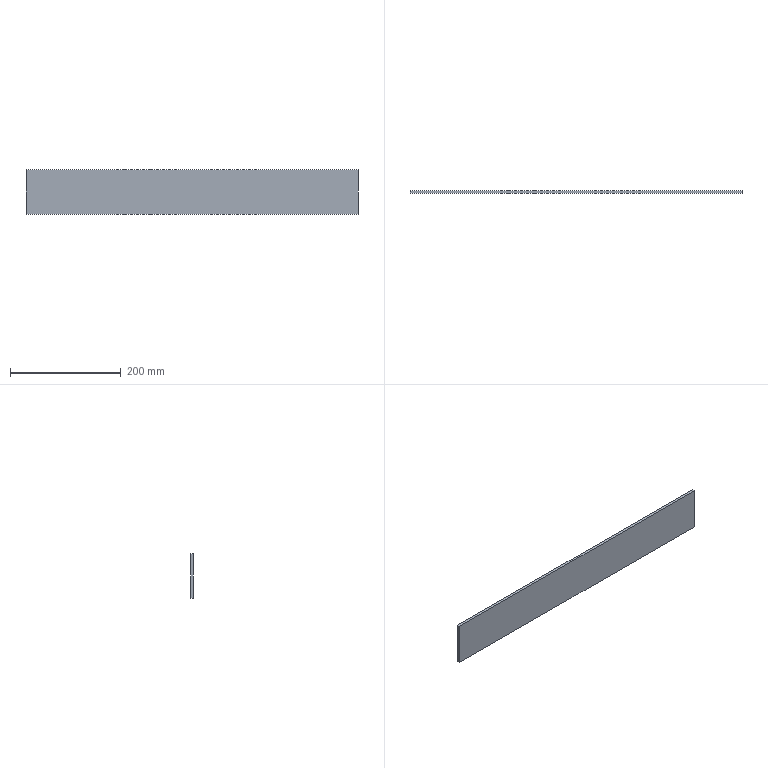Component | SolidWorks | CoverPlate6-1 | 1 solid | 6 faces | box 600 x 5 x 80 mm | volume 240000 mm3 | plane 6
build123d program:
from build123d import *

# Parameters (mm, degrees)
SKETCH1_W      = 600
SKETCH1_H      = 80
EXTRUDE1_DEPTH = 5


with BuildPart() as part:
    # Sketch1 → Extrude1 (new body)
    with BuildSketch(Plane.XY):
        Rectangle(SKETCH1_W, SKETCH1_H)
    extrude(amount=EXTRUDE1_DEPTH)


solid = part.part

# Placed as in the assembly
solid = solid.moved(Location((15, 95, -60), (90, 0, 0)))
STEP:
#1=COLOUR_RGB('',0.7922,0.8196,0.9333);
#2=FILL_AREA_STYLE_COLOUR('',#1);
#3=FILL_AREA_STYLE('',(#2));
#4=SURFACE_STYLE_FILL_AREA(#3);
#5=SURFACE_SIDE_STYLE('',(#4));
#6=SURFACE_STYLE_USAGE(.BOTH.,#5);
#7=PRESENTATION_STYLE_ASSIGNMENT((#6));
#8=CARTESIAN_POINT('',(12.402,3.543,-0.7874));
#9=VERTEX_POINT('',#8);
#10=CARTESIAN_POINT('',(12.402,3.543,-3.937));
#11=VERTEX_POINT('',#10);
#12=CARTESIAN_POINT('',(12.402,3.543,-3.937));
#13=DIRECTION('',(0.,0.,-1.));
#14=VECTOR('',#13,39.37);
#15=LINE('',#12,#14);
#16=EDGE_CURVE('',#9,#11,#15,.T.);
#17=ORIENTED_EDGE('',*,*,#16,.T.);
#18=CARTESIAN_POINT('',(12.402,3.74,-3.937));
#19=VERTEX_POINT('',#18);
#20=CARTESIAN_POINT('',(12.402,3.74,-3.937));
#21=DIRECTION('',(0.,-1.,0.));
#22=VECTOR('',#21,39.37);
#23=LINE('',#20,#22);
#24=EDGE_CURVE('',#19,#11,#23,.T.);
#25=ORIENTED_EDGE('',*,*,#24,.F.);
#26=CARTESIAN_POINT('',(12.402,3.74,-0.7874));
#27=VERTEX_POINT('',#26);
#28=CARTESIAN_POINT('',(12.402,3.74,-3.937));
#29=DIRECTION('',(0.,0.,-1.));
#30=VECTOR('',#29,39.37);
#31=LINE('',#28,#30);
#32=EDGE_CURVE('',#27,#19,#31,.T.);
#33=ORIENTED_EDGE('',*,*,#32,.F.);
#34=CARTESIAN_POINT('',(12.402,3.74,-0.7874));
#35=DIRECTION('',(0.,-1.,0.));
#36=VECTOR('',#35,39.37);
#37=LINE('',#34,#36);
#38=EDGE_CURVE('',#27,#9,#37,.T.);
#39=ORIENTED_EDGE('',*,*,#38,.T.);
#40=EDGE_LOOP('',(#17,#25,#33,#39));
#41=FACE_OUTER_BOUND('',#40,.T.);
#42=CARTESIAN_POINT('',(12.402,3.74,-3.937));
#43=DIRECTION('',(-1.,0.,0.));
#44=DIRECTION('',(0.,1.,0.));
#45=AXIS2_PLACEMENT_3D('',#42,#43,#44);
#46=PLANE('',#45);
#47=ADVANCED_FACE('',(#41),#46,.F.);
#48=CARTESIAN_POINT('',(-11.22,3.543,-3.937));
#49=VERTEX_POINT('',#48);
#50=CARTESIAN_POINT('',(-11.22,3.543,-3.937));
#51=DIRECTION('',(-1.,0.,0.));
#52=VECTOR('',#51,39.37);
#53=LINE('',#50,#52);
#54=EDGE_CURVE('',#11,#49,#53,.T.);
#55=ORIENTED_EDGE('',*,*,#54,.T.);
#56=CARTESIAN_POINT('',(-11.22,3.74,-3.937));
#57=VERTEX_POINT('',#56);
#58=CARTESIAN_POINT('',(-11.22,3.74,-3.937));
#59=DIRECTION('',(0.,-1.,0.));
#60=VECTOR('',#59,39.37);
#61=LINE('',#58,#60);
#62=EDGE_CURVE('',#57,#49,#61,.T.);
#63=ORIENTED_EDGE('',*,*,#62,.F.);
#64=CARTESIAN_POINT('',(-11.22,3.74,-3.937));
#65=DIRECTION('',(-1.,0.,0.));
#66=VECTOR('',#65,39.37);
#67=LINE('',#64,#66);
#68=EDGE_CURVE('',#19,#57,#67,.T.);
#69=ORIENTED_EDGE('',*,*,#68,.F.);
#70=ORIENTED_EDGE('',*,*,#24,.T.);
#71=EDGE_LOOP('',(#55,#63,#69,#70));
#72=FACE_OUTER_BOUND('',#71,.T.);
#73=CARTESIAN_POINT('',(-11.22,3.74,-3.937));
#74=DIRECTION('',(0.,0.,1.));
#75=DIRECTION('',(0.,-1.,0.));
#76=AXIS2_PLACEMENT_3D('',#73,#74,#75);
#77=PLANE('',#76);
#78=ADVANCED_FACE('',(#72),#77,.F.);
#79=CARTESIAN_POINT('',(-11.22,3.543,-0.7874));
#80=VERTEX_POINT('',#79);
#81=CARTESIAN_POINT('',(-11.22,3.543,-3.937));
#82=DIRECTION('',(0.,0.,1.));
#83=VECTOR('',#82,39.37);
#84=LINE('',#81,#83);
#85=EDGE_CURVE('',#49,#80,#84,.T.);
#86=ORIENTED_EDGE('',*,*,#85,.T.);
#87=CARTESIAN_POINT('',(-11.22,3.74,-0.7874));
#88=VERTEX_POINT('',#87);
#89=CARTESIAN_POINT('',(-11.22,3.74,-0.7874));
#90=DIRECTION('',(0.,-1.,0.));
#91=VECTOR('',#90,39.37);
#92=LINE('',#89,#91);
#93=EDGE_CURVE('',#88,#80,#92,.T.);
#94=ORIENTED_EDGE('',*,*,#93,.F.);
#95=CARTESIAN_POINT('',(-11.22,3.74,-3.937));
#96=DIRECTION('',(0.,0.,1.));
#97=VECTOR('',#96,39.37);
#98=LINE('',#95,#97);
#99=EDGE_CURVE('',#57,#88,#98,.T.);
#100=ORIENTED_EDGE('',*,*,#99,.F.);
#101=ORIENTED_EDGE('',*,*,#62,.T.);
#102=EDGE_LOOP('',(#86,#94,#100,#101));
#103=FACE_OUTER_BOUND('',#102,.T.);
#104=CARTESIAN_POINT('',(-11.22,3.74,-3.937));
#105=DIRECTION('',(1.,0.,0.));
#106=DIRECTION('',(0.,-1.,0.));
#107=AXIS2_PLACEMENT_3D('',#104,#105,#106);
#108=PLANE('',#107);
#109=ADVANCED_FACE('',(#103),#108,.F.);
#110=CARTESIAN_POINT('',(-11.22,3.543,-0.7874));
#111=DIRECTION('',(1.,0.,0.));
#112=VECTOR('',#111,39.37);
#113=LINE('',#110,#112);
#114=EDGE_CURVE('',#80,#9,#113,.T.);
#115=ORIENTED_EDGE('',*,*,#114,.T.);
#116=ORIENTED_EDGE('',*,*,#38,.F.);
#117=CARTESIAN_POINT('',(-11.22,3.74,-0.7874));
#118=DIRECTION('',(1.,0.,0.));
#119=VECTOR('',#118,39.37);
#120=LINE('',#117,#119);
#121=EDGE_CURVE('',#88,#27,#120,.T.);
#122=ORIENTED_EDGE('',*,*,#121,.F.);
#123=ORIENTED_EDGE('',*,*,#93,.T.);
#124=EDGE_LOOP('',(#115,#116,#122,#123));
#125=FACE_OUTER_BOUND('',#124,.T.);
#126=CARTESIAN_POINT('',(-11.22,3.74,-0.7874));
#127=DIRECTION('',(0.,0.,-1.));
#128=DIRECTION('',(0.,1.,0.));
#129=AXIS2_PLACEMENT_3D('',#126,#127,#128);
#130=PLANE('',#129);
#131=ADVANCED_FACE('',(#125),#130,.F.);
#132=ORIENTED_EDGE('',*,*,#32,.T.);
#133=ORIENTED_EDGE('',*,*,#68,.T.);
#134=ORIENTED_EDGE('',*,*,#99,.T.);
#135=ORIENTED_EDGE('',*,*,#121,.T.);
#136=EDGE_LOOP('',(#132,#133,#134,#135));
#137=FACE_OUTER_BOUND('',#136,.T.);
#138=CARTESIAN_POINT('',(0.5906,3.74,-2.362));
#139=DIRECTION('',(0.,1.,0.));
#140=DIRECTION('',(1.,0.,0.));
#141=AXIS2_PLACEMENT_3D('',#138,#139,#140);
#142=PLANE('',#141);
#143=ADVANCED_FACE('',(#137),#142,.T.);
#144=ORIENTED_EDGE('',*,*,#16,.F.);
#145=ORIENTED_EDGE('',*,*,#114,.F.);
#146=ORIENTED_EDGE('',*,*,#85,.F.);
#147=ORIENTED_EDGE('',*,*,#54,.F.);
#148=EDGE_LOOP('',(#144,#145,#146,#147));
#149=FACE_OUTER_BOUND('',#148,.T.);
#150=CARTESIAN_POINT('',(0.5906,3.543,-2.362));
#151=DIRECTION('',(0.,1.,0.));
#152=DIRECTION('',(1.,0.,0.));
#153=AXIS2_PLACEMENT_3D('',#150,#151,#152);
#154=PLANE('',#153);
#155=ADVANCED_FACE('',(#149),#154,.F.);
#156=CLOSED_SHELL('',(#47,#78,#109,#131,#143,#155));
#157=MANIFOLD_SOLID_BREP('',#156);
#158=STYLED_ITEM('',(#7),#157);
#159=(LENGTH_UNIT()NAMED_UNIT(*)SI_UNIT($,.METRE.));
#160=LENGTH_MEASURE_WITH_UNIT(LENGTH_MEASURE(0.0254),#159);
#161=DIMENSIONAL_EXPONENTS(1.,0.,0.,0.,0.,0.,0.);
#162=(CONVERSION_BASED_UNIT('',#160)LENGTH_UNIT()NAMED_UNIT(#161));
#163=UNCERTAINTY_MEASURE_WITH_UNIT(LENGTH_MEASURE(0.00001),#162,'','');
#164=(NAMED_UNIT(*)PLANE_ANGLE_UNIT()SI_UNIT($,.RADIAN.));
#165=(NAMED_UNIT(*)SI_UNIT($,.STERADIAN.)SOLID_ANGLE_UNIT());
#166=(GEOMETRIC_REPRESENTATION_CONTEXT(3)GLOBAL_UNCERTAINTY_ASSIGNED_CONTEXT((#163))GLOBAL_UNIT_ASSIGNED_CONTEXT((#162,#164,#165))REPRESENTATION_CONTEXT('',''));
#167=MECHANICAL_DESIGN_GEOMETRIC_PRESENTATION_REPRESENTATION('',(#158),#166);
#168=PRESENTATION_LAYER_ASSIGNMENT('','',(#158));
#169=CARTESIAN_POINT('',(0.,0.,0.));
#170=DIRECTION('',(0.,0.,1.));
#171=DIRECTION('',(1.,0.,0.));
#172=AXIS2_PLACEMENT_3D('',#169,#170,#171);
#173=(LENGTH_UNIT()NAMED_UNIT(*)SI_UNIT($,.METRE.));
#174=LENGTH_MEASURE_WITH_UNIT(LENGTH_MEASURE(0.0254),#173);
#175=DIMENSIONAL_EXPONENTS(1.,0.,0.,0.,0.,0.,0.);
#176=(CONVERSION_BASED_UNIT('',#174)LENGTH_UNIT()NAMED_UNIT(#175));
#177=UNCERTAINTY_MEASURE_WITH_UNIT(LENGTH_MEASURE(0.00001),#176,'','');
#178=(NAMED_UNIT(*)PLANE_ANGLE_UNIT()SI_UNIT($,.RADIAN.));
#179=(NAMED_UNIT(*)SI_UNIT($,.STERADIAN.)SOLID_ANGLE_UNIT());
#180=(GEOMETRIC_REPRESENTATION_CONTEXT(3)GLOBAL_UNCERTAINTY_ASSIGNED_CONTEXT((#177))GLOBAL_UNIT_ASSIGNED_CONTEXT((#176,#178,#179))REPRESENTATION_CONTEXT('',''));
#181=ADVANCED_BREP_SHAPE_REPRESENTATION('',(#157,#172),#180);